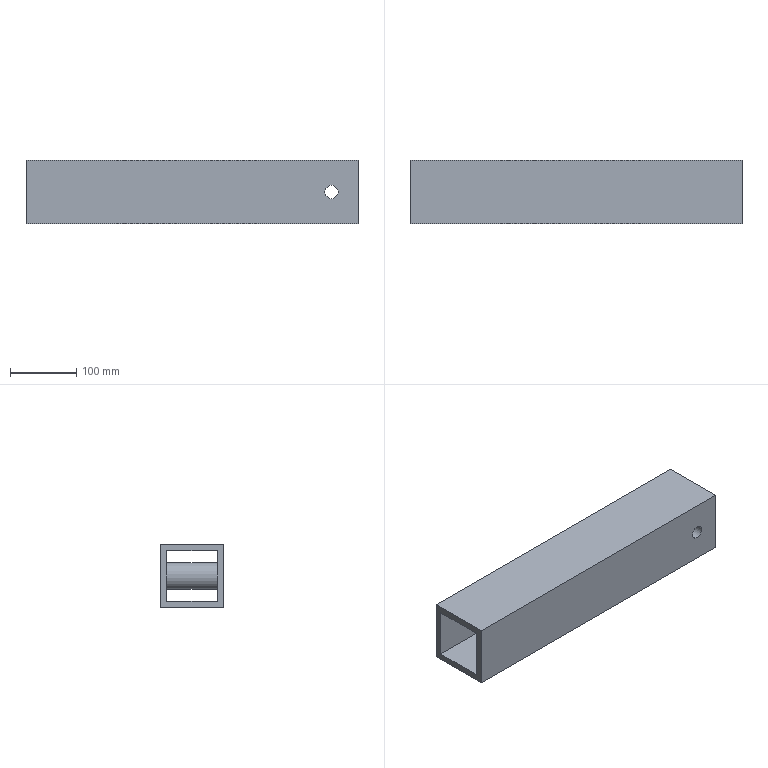Component | NX | TELESCOPIC_ROD | 1 solid | 12 faces | box 500 x 96 x 96 mm | volume 1785345 mm3 | plane 10 | cylinder 2 | commonest cylinder face diameters 20 x1 40 x1
STEP:
#1=CARTESIAN_POINT('',(0.,0.,0.));
#2=DIRECTION('',(0.,0.,1.));
#3=DIRECTION('',(1.,0.,0.));
#4=AXIS2_PLACEMENT_3D('',#1,#2,#3);
#5=CARTESIAN_POINT('',(1094.,88.,-44.));
#6=VERTEX_POINT('',#5);
#7=CARTESIAN_POINT('',(1094.,88.,-120.));
#8=VERTEX_POINT('',#7);
#9=CARTESIAN_POINT('',(1094.,88.,-34.));
#10=DIRECTION('',(0.,-0.,-1.));
#11=VECTOR('',#10,1.);
#12=LINE('',#9,#11);
#13=CARTESIAN_POINT('',(1094.,174.,-34.));
#14=DIRECTION('',(-1.,0.,0.));
#15=DIRECTION('',(0.,-1.,0.));
#16=AXIS2_PLACEMENT_3D('',#13,#14,#15);
#17=PLANE('',#16);
#18=CARTESIAN_POINT('',(86.,0.));
#19=DIRECTION('',(0.,-1.));
#20=VECTOR('',#19,1.);
#21=LINE('',#18,#20);
#22=(GEOMETRIC_REPRESENTATION_CONTEXT(2)PARAMETRIC_REPRESENTATION_CONTEXT()REPRESENTATION_CONTEXT('',''));
#23=DEFINITIONAL_REPRESENTATION('',(#21),#22);
#24=PCURVE('',#17,#23);
#25=CARTESIAN_POINT('',(594.,88.,-34.));
#26=DIRECTION('',(0.,-1.,0.));
#27=DIRECTION('',(0.,-0.,-1.));
#28=AXIS2_PLACEMENT_3D('',#25,#26,#27);
#29=PLANE('',#28);
#30=CARTESIAN_POINT('',(0.,500.));
#31=DIRECTION('',(1.,0.));
#32=VECTOR('',#31,1.);
#33=LINE('',#30,#32);
#34=(GEOMETRIC_REPRESENTATION_CONTEXT(2)PARAMETRIC_REPRESENTATION_CONTEXT()REPRESENTATION_CONTEXT('',''));
#35=DEFINITIONAL_REPRESENTATION('',(#33),#34);
#36=PCURVE('',#29,#35);
#37=SURFACE_CURVE('',#12,(#24,#36),.PCURVE_S1.);
#38=EDGE_CURVE('',#6,#8,#37,.T.);
#39=ORIENTED_EDGE('',*,*,#38,.F.);
#40=CARTESIAN_POINT('',(1094.,164.,-44.));
#41=VERTEX_POINT('',#40);
#42=CARTESIAN_POINT('',(1094.,174.,-44.));
#43=DIRECTION('',(0.,-1.,0.));
#44=VECTOR('',#43,1.);
#45=LINE('',#42,#44);
#46=CARTESIAN_POINT('',(0.,-10.));
#47=DIRECTION('',(1.,0.));
#48=VECTOR('',#47,1.);
#49=LINE('',#46,#48);
#50=(GEOMETRIC_REPRESENTATION_CONTEXT(2)PARAMETRIC_REPRESENTATION_CONTEXT()REPRESENTATION_CONTEXT('',''));
#51=DEFINITIONAL_REPRESENTATION('',(#49),#50);
#52=PCURVE('',#17,#51);
#53=CARTESIAN_POINT('',(594.,174.,-44.));
#54=DIRECTION('',(0.,0.,1.));
#55=DIRECTION('',(1.,0.,0.));
#56=AXIS2_PLACEMENT_3D('',#53,#54,#55);
#57=PLANE('',#56);
#58=CARTESIAN_POINT('',(500.,0.));
#59=DIRECTION('',(0.,-1.));
#60=VECTOR('',#59,1.);
#61=LINE('',#58,#60);
#62=(GEOMETRIC_REPRESENTATION_CONTEXT(2)PARAMETRIC_REPRESENTATION_CONTEXT()REPRESENTATION_CONTEXT('',''));
#63=DEFINITIONAL_REPRESENTATION('',(#61),#62);
#64=PCURVE('',#57,#63);
#65=SURFACE_CURVE('',#45,(#52,#64),.PCURVE_S1.);
#66=EDGE_CURVE('',#41,#6,#65,.T.);
#67=ORIENTED_EDGE('',*,*,#66,.F.);
#68=CARTESIAN_POINT('',(1094.,164.,-120.));
#69=VERTEX_POINT('',#68);
#70=CARTESIAN_POINT('',(1094.,164.,-130.));
#71=DIRECTION('',(0.,-0.,1.));
#72=VECTOR('',#71,1.);
#73=LINE('',#70,#72);
#74=CARTESIAN_POINT('',(10.,-96.));
#75=DIRECTION('',(0.,1.));
#76=VECTOR('',#75,1.);
#77=LINE('',#74,#76);
#78=(GEOMETRIC_REPRESENTATION_CONTEXT(2)PARAMETRIC_REPRESENTATION_CONTEXT()REPRESENTATION_CONTEXT('',''));
#79=DEFINITIONAL_REPRESENTATION('',(#77),#78);
#80=PCURVE('',#17,#79);
#81=CARTESIAN_POINT('',(594.,164.,-130.));
#82=DIRECTION('',(0.,1.,0.));
#83=DIRECTION('',(0.,-0.,1.));
#84=AXIS2_PLACEMENT_3D('',#81,#82,#83);
#85=PLANE('',#84);
#86=CARTESIAN_POINT('',(0.,500.));
#87=DIRECTION('',(1.,0.));
#88=VECTOR('',#87,1.);
#89=LINE('',#86,#88);
#90=(GEOMETRIC_REPRESENTATION_CONTEXT(2)PARAMETRIC_REPRESENTATION_CONTEXT()REPRESENTATION_CONTEXT('',''));
#91=DEFINITIONAL_REPRESENTATION('',(#89),#90);
#92=PCURVE('',#85,#91);
#93=SURFACE_CURVE('',#73,(#80,#92),.PCURVE_S1.);
#94=EDGE_CURVE('',#69,#41,#93,.T.);
#95=ORIENTED_EDGE('',*,*,#94,.F.);
#96=CARTESIAN_POINT('',(1094.,78.,-120.));
#97=DIRECTION('',(0.,1.,0.));
#98=VECTOR('',#97,1.);
#99=LINE('',#96,#98);
#100=CARTESIAN_POINT('',(96.,-86.));
#101=DIRECTION('',(-1.,0.));
#102=VECTOR('',#101,1.);
#103=LINE('',#100,#102);
#104=(GEOMETRIC_REPRESENTATION_CONTEXT(2)PARAMETRIC_REPRESENTATION_CONTEXT()REPRESENTATION_CONTEXT('',''));
#105=DEFINITIONAL_REPRESENTATION('',(#103),#104);
#106=PCURVE('',#17,#105);
#107=CARTESIAN_POINT('',(594.,78.,-120.));
#108=DIRECTION('',(0.,0.,-1.));
#109=DIRECTION('',(-1.,0.,0.));
#110=AXIS2_PLACEMENT_3D('',#107,#108,#109);
#111=PLANE('',#110);
#112=CARTESIAN_POINT('',(-500.,0.));
#113=DIRECTION('',(0.,1.));
#114=VECTOR('',#113,1.);
#115=LINE('',#112,#114);
#116=(GEOMETRIC_REPRESENTATION_CONTEXT(2)PARAMETRIC_REPRESENTATION_CONTEXT()REPRESENTATION_CONTEXT('',''));
#117=DEFINITIONAL_REPRESENTATION('',(#115),#116);
#118=PCURVE('',#111,#117);
#119=SURFACE_CURVE('',#99,(#106,#118),.PCURVE_S1.);
#120=EDGE_CURVE('',#8,#69,#119,.T.);
#121=ORIENTED_EDGE('',*,*,#120,.F.);
#122=EDGE_LOOP('',(#39,#67,#95,#121));
#123=FACE_BOUND('',#122,.T.);
#124=CARTESIAN_POINT('',(1094.,174.,-34.));
#125=VERTEX_POINT('',#124);
#126=CARTESIAN_POINT('',(1094.,78.,-34.));
#127=VERTEX_POINT('',#126);
#128=CARTESIAN_POINT('',(1094.,174.,-34.));
#129=DIRECTION('',(0.,-1.,0.));
#130=VECTOR('',#129,1.);
#131=LINE('',#128,#130);
#132=CARTESIAN_POINT('',(0.,0.));
#133=DIRECTION('',(1.,0.));
#134=VECTOR('',#133,1.);
#135=LINE('',#132,#134);
#136=(GEOMETRIC_REPRESENTATION_CONTEXT(2)PARAMETRIC_REPRESENTATION_CONTEXT()REPRESENTATION_CONTEXT('',''));
#137=DEFINITIONAL_REPRESENTATION('',(#135),#136);
#138=PCURVE('',#17,#137);
#139=CARTESIAN_POINT('',(594.,174.,-34.));
#140=DIRECTION('',(0.,0.,1.));
#141=DIRECTION('',(1.,0.,0.));
#142=AXIS2_PLACEMENT_3D('',#139,#140,#141);
#143=PLANE('',#142);
#144=CARTESIAN_POINT('',(500.,0.));
#145=DIRECTION('',(0.,-1.));
#146=VECTOR('',#145,1.);
#147=LINE('',#144,#146);
#148=(GEOMETRIC_REPRESENTATION_CONTEXT(2)PARAMETRIC_REPRESENTATION_CONTEXT()REPRESENTATION_CONTEXT('',''));
#149=DEFINITIONAL_REPRESENTATION('',(#147),#148);
#150=PCURVE('',#143,#149);
#151=SURFACE_CURVE('',#131,(#138,#150),.PCURVE_S1.);
#152=EDGE_CURVE('',#125,#127,#151,.T.);
#153=ORIENTED_EDGE('',*,*,#152,.T.);
#154=CARTESIAN_POINT('',(1094.,78.,-130.));
#155=VERTEX_POINT('',#154);
#156=CARTESIAN_POINT('',(1094.,78.,-34.));
#157=DIRECTION('',(0.,-0.,-1.));
#158=VECTOR('',#157,1.);
#159=LINE('',#156,#158);
#160=CARTESIAN_POINT('',(96.,0.));
#161=DIRECTION('',(0.,-1.));
#162=VECTOR('',#161,1.);
#163=LINE('',#160,#162);
#164=(GEOMETRIC_REPRESENTATION_CONTEXT(2)PARAMETRIC_REPRESENTATION_CONTEXT()REPRESENTATION_CONTEXT('',''));
#165=DEFINITIONAL_REPRESENTATION('',(#163),#164);
#166=PCURVE('',#17,#165);
#167=CARTESIAN_POINT('',(594.,78.,-34.));
#168=DIRECTION('',(0.,-1.,0.));
#169=DIRECTION('',(0.,-0.,-1.));
#170=AXIS2_PLACEMENT_3D('',#167,#168,#169);
#171=PLANE('',#170);
#172=CARTESIAN_POINT('',(0.,500.));
#173=DIRECTION('',(1.,0.));
#174=VECTOR('',#173,1.);
#175=LINE('',#172,#174);
#176=(GEOMETRIC_REPRESENTATION_CONTEXT(2)PARAMETRIC_REPRESENTATION_CONTEXT()REPRESENTATION_CONTEXT('',''));
#177=DEFINITIONAL_REPRESENTATION('',(#175),#176);
#178=PCURVE('',#171,#177);
#179=SURFACE_CURVE('',#159,(#166,#178),.PCURVE_S1.);
#180=EDGE_CURVE('',#127,#155,#179,.T.);
#181=ORIENTED_EDGE('',*,*,#180,.T.);
#182=CARTESIAN_POINT('',(1094.,174.,-130.));
#183=VERTEX_POINT('',#182);
#184=CARTESIAN_POINT('',(1094.,78.,-130.));
#185=DIRECTION('',(0.,1.,0.));
#186=VECTOR('',#185,1.);
#187=LINE('',#184,#186);
#188=CARTESIAN_POINT('',(96.,-96.));
#189=DIRECTION('',(-1.,0.));
#190=VECTOR('',#189,1.);
#191=LINE('',#188,#190);
#192=(GEOMETRIC_REPRESENTATION_CONTEXT(2)PARAMETRIC_REPRESENTATION_CONTEXT()REPRESENTATION_CONTEXT('',''));
#193=DEFINITIONAL_REPRESENTATION('',(#191),#192);
#194=PCURVE('',#17,#193);
#195=CARTESIAN_POINT('',(594.,78.,-130.));
#196=DIRECTION('',(0.,0.,-1.));
#197=DIRECTION('',(-1.,0.,0.));
#198=AXIS2_PLACEMENT_3D('',#195,#196,#197);
#199=PLANE('',#198);
#200=CARTESIAN_POINT('',(-500.,0.));
#201=DIRECTION('',(0.,1.));
#202=VECTOR('',#201,1.);
#203=LINE('',#200,#202);
#204=(GEOMETRIC_REPRESENTATION_CONTEXT(2)PARAMETRIC_REPRESENTATION_CONTEXT()REPRESENTATION_CONTEXT('',''));
#205=DEFINITIONAL_REPRESENTATION('',(#203),#204);
#206=PCURVE('',#199,#205);
#207=SURFACE_CURVE('',#187,(#194,#206),.PCURVE_S1.);
#208=EDGE_CURVE('',#155,#183,#207,.T.);
#209=ORIENTED_EDGE('',*,*,#208,.T.);
#210=CARTESIAN_POINT('',(1094.,174.,-130.));
#211=DIRECTION('',(0.,-0.,1.));
#212=VECTOR('',#211,1.);
#213=LINE('',#210,#212);
#214=CARTESIAN_POINT('',(0.,-96.));
#215=DIRECTION('',(0.,1.));
#216=VECTOR('',#215,1.);
#217=LINE('',#214,#216);
#218=(GEOMETRIC_REPRESENTATION_CONTEXT(2)PARAMETRIC_REPRESENTATION_CONTEXT()REPRESENTATION_CONTEXT('',''));
#219=DEFINITIONAL_REPRESENTATION('',(#217),#218);
#220=PCURVE('',#17,#219);
#221=CARTESIAN_POINT('',(594.,174.,-130.));
#222=DIRECTION('',(0.,1.,0.));
#223=DIRECTION('',(0.,-0.,1.));
#224=AXIS2_PLACEMENT_3D('',#221,#222,#223);
#225=PLANE('',#224);
#226=CARTESIAN_POINT('',(0.,500.));
#227=DIRECTION('',(1.,0.));
#228=VECTOR('',#227,1.);
#229=LINE('',#226,#228);
#230=(GEOMETRIC_REPRESENTATION_CONTEXT(2)PARAMETRIC_REPRESENTATION_CONTEXT()REPRESENTATION_CONTEXT('',''));
#231=DEFINITIONAL_REPRESENTATION('',(#229),#230);
#232=PCURVE('',#225,#231);
#233=SURFACE_CURVE('',#213,(#220,#232),.PCURVE_S1.);
#234=EDGE_CURVE('',#183,#125,#233,.T.);
#235=ORIENTED_EDGE('',*,*,#234,.T.);
#236=EDGE_LOOP('',(#153,#181,#209,#235));
#237=FACE_BOUND('',#236,.T.);
#238=ADVANCED_FACE('',(#123,#237),#17,.F.);
#239=CARTESIAN_POINT('',(594.,88.,-44.));
#240=VERTEX_POINT('',#239);
#241=CARTESIAN_POINT('',(594.,88.,-120.));
#242=VERTEX_POINT('',#241);
#243=CARTESIAN_POINT('',(594.,88.,-34.));
#244=DIRECTION('',(0.,-0.,-1.));
#245=VECTOR('',#244,1.);
#246=LINE('',#243,#245);
#247=CARTESIAN_POINT('',(594.,78.,-130.));
#248=DIRECTION('',(-1.,0.,0.));
#249=DIRECTION('',(0.,1.,0.));
#250=AXIS2_PLACEMENT_3D('',#247,#248,#249);
#251=PLANE('',#250);
#252=CARTESIAN_POINT('',(10.,-96.));
#253=DIRECTION('',(-0.,1.));
#254=VECTOR('',#253,1.);
#255=LINE('',#252,#254);
#256=(GEOMETRIC_REPRESENTATION_CONTEXT(2)PARAMETRIC_REPRESENTATION_CONTEXT()REPRESENTATION_CONTEXT('',''));
#257=DEFINITIONAL_REPRESENTATION('',(#255),#256);
#258=PCURVE('',#251,#257);
#259=CARTESIAN_POINT('',(0.,0.));
#260=DIRECTION('',(1.,0.));
#261=VECTOR('',#260,1.);
#262=LINE('',#259,#261);
#263=(GEOMETRIC_REPRESENTATION_CONTEXT(2)PARAMETRIC_REPRESENTATION_CONTEXT()REPRESENTATION_CONTEXT('',''));
#264=DEFINITIONAL_REPRESENTATION('',(#262),#263);
#265=PCURVE('',#29,#264);
#266=SURFACE_CURVE('',#246,(#258,#265),.PCURVE_S1.);
#267=EDGE_CURVE('',#240,#242,#266,.T.);
#268=ORIENTED_EDGE('',*,*,#267,.T.);
#269=CARTESIAN_POINT('',(594.,164.,-120.));
#270=VERTEX_POINT('',#269);
#271=CARTESIAN_POINT('',(594.,78.,-120.));
#272=DIRECTION('',(0.,1.,0.));
#273=VECTOR('',#272,1.);
#274=LINE('',#271,#273);
#275=CARTESIAN_POINT('',(0.,-10.));
#276=DIRECTION('',(1.,0.));
#277=VECTOR('',#276,1.);
#278=LINE('',#275,#277);
#279=(GEOMETRIC_REPRESENTATION_CONTEXT(2)PARAMETRIC_REPRESENTATION_CONTEXT()REPRESENTATION_CONTEXT('',''));
#280=DEFINITIONAL_REPRESENTATION('',(#278),#279);
#281=PCURVE('',#251,#280);
#282=CARTESIAN_POINT('',(0.,0.));
#283=DIRECTION('',(0.,1.));
#284=VECTOR('',#283,1.);
#285=LINE('',#282,#284);
#286=(GEOMETRIC_REPRESENTATION_CONTEXT(2)PARAMETRIC_REPRESENTATION_CONTEXT()REPRESENTATION_CONTEXT('',''));
#287=DEFINITIONAL_REPRESENTATION('',(#285),#286);
#288=PCURVE('',#111,#287);
#289=SURFACE_CURVE('',#274,(#281,#288),.PCURVE_S1.);
#290=EDGE_CURVE('',#242,#270,#289,.T.);
#291=ORIENTED_EDGE('',*,*,#290,.T.);
#292=CARTESIAN_POINT('',(594.,164.,-44.));
#293=VERTEX_POINT('',#292);
#294=CARTESIAN_POINT('',(594.,164.,-130.));
#295=DIRECTION('',(0.,-0.,1.));
#296=VECTOR('',#295,1.);
#297=LINE('',#294,#296);
#298=CARTESIAN_POINT('',(86.,0.));
#299=DIRECTION('',(-0.,-1.));
#300=VECTOR('',#299,1.);
#301=LINE('',#298,#300);
#302=(GEOMETRIC_REPRESENTATION_CONTEXT(2)PARAMETRIC_REPRESENTATION_CONTEXT()REPRESENTATION_CONTEXT('',''));
#303=DEFINITIONAL_REPRESENTATION('',(#301),#302);
#304=PCURVE('',#251,#303);
#305=CARTESIAN_POINT('',(0.,0.));
#306=DIRECTION('',(1.,0.));
#307=VECTOR('',#306,1.);
#308=LINE('',#305,#307);
#309=(GEOMETRIC_REPRESENTATION_CONTEXT(2)PARAMETRIC_REPRESENTATION_CONTEXT()REPRESENTATION_CONTEXT('',''));
#310=DEFINITIONAL_REPRESENTATION('',(#308),#309);
#311=PCURVE('',#85,#310);
#312=SURFACE_CURVE('',#297,(#304,#311),.PCURVE_S1.);
#313=EDGE_CURVE('',#270,#293,#312,.T.);
#314=ORIENTED_EDGE('',*,*,#313,.T.);
#315=CARTESIAN_POINT('',(594.,174.,-44.));
#316=DIRECTION('',(0.,-1.,0.));
#317=VECTOR('',#316,1.);
#318=LINE('',#315,#317);
#319=CARTESIAN_POINT('',(96.,-86.));
#320=DIRECTION('',(-1.,0.));
#321=VECTOR('',#320,1.);
#322=LINE('',#319,#321);
#323=(GEOMETRIC_REPRESENTATION_CONTEXT(2)PARAMETRIC_REPRESENTATION_CONTEXT()REPRESENTATION_CONTEXT('',''));
#324=DEFINITIONAL_REPRESENTATION('',(#322),#323);
#325=PCURVE('',#251,#324);
#326=CARTESIAN_POINT('',(0.,0.));
#327=DIRECTION('',(0.,-1.));
#328=VECTOR('',#327,1.);
#329=LINE('',#326,#328);
#330=(GEOMETRIC_REPRESENTATION_CONTEXT(2)PARAMETRIC_REPRESENTATION_CONTEXT()REPRESENTATION_CONTEXT('',''));
#331=DEFINITIONAL_REPRESENTATION('',(#329),#330);
#332=PCURVE('',#57,#331);
#333=SURFACE_CURVE('',#318,(#325,#332),.PCURVE_S1.);
#334=EDGE_CURVE('',#293,#240,#333,.T.);
#335=ORIENTED_EDGE('',*,*,#334,.T.);
#336=EDGE_LOOP('',(#268,#291,#314,#335));
#337=FACE_BOUND('',#336,.T.);
#338=CARTESIAN_POINT('',(594.,78.,-130.));
#339=VERTEX_POINT('',#338);
#340=CARTESIAN_POINT('',(594.,174.,-130.));
#341=VERTEX_POINT('',#340);
#342=CARTESIAN_POINT('',(594.,78.,-130.));
#343=DIRECTION('',(0.,1.,0.));
#344=VECTOR('',#343,1.);
#345=LINE('',#342,#344);
#346=CARTESIAN_POINT('',(0.,0.));
#347=DIRECTION('',(1.,0.));
#348=VECTOR('',#347,1.);
#349=LINE('',#346,#348);
#350=(GEOMETRIC_REPRESENTATION_CONTEXT(2)PARAMETRIC_REPRESENTATION_CONTEXT()REPRESENTATION_CONTEXT('',''));
#351=DEFINITIONAL_REPRESENTATION('',(#349),#350);
#352=PCURVE('',#251,#351);
#353=CARTESIAN_POINT('',(0.,0.));
#354=DIRECTION('',(0.,1.));
#355=VECTOR('',#354,1.);
#356=LINE('',#353,#355);
#357=(GEOMETRIC_REPRESENTATION_CONTEXT(2)PARAMETRIC_REPRESENTATION_CONTEXT()REPRESENTATION_CONTEXT('',''));
#358=DEFINITIONAL_REPRESENTATION('',(#356),#357);
#359=PCURVE('',#199,#358);
#360=SURFACE_CURVE('',#345,(#352,#359),.PCURVE_S1.);
#361=EDGE_CURVE('',#339,#341,#360,.T.);
#362=ORIENTED_EDGE('',*,*,#361,.F.);
#363=CARTESIAN_POINT('',(594.,78.,-34.));
#364=VERTEX_POINT('',#363);
#365=CARTESIAN_POINT('',(594.,78.,-34.));
#366=DIRECTION('',(0.,-0.,-1.));
#367=VECTOR('',#366,1.);
#368=LINE('',#365,#367);
#369=CARTESIAN_POINT('',(0.,-96.));
#370=DIRECTION('',(-0.,1.));
#371=VECTOR('',#370,1.);
#372=LINE('',#369,#371);
#373=(GEOMETRIC_REPRESENTATION_CONTEXT(2)PARAMETRIC_REPRESENTATION_CONTEXT()REPRESENTATION_CONTEXT('',''));
#374=DEFINITIONAL_REPRESENTATION('',(#372),#373);
#375=PCURVE('',#251,#374);
#376=CARTESIAN_POINT('',(0.,0.));
#377=DIRECTION('',(1.,0.));
#378=VECTOR('',#377,1.);
#379=LINE('',#376,#378);
#380=(GEOMETRIC_REPRESENTATION_CONTEXT(2)PARAMETRIC_REPRESENTATION_CONTEXT()REPRESENTATION_CONTEXT('',''));
#381=DEFINITIONAL_REPRESENTATION('',(#379),#380);
#382=PCURVE('',#171,#381);
#383=SURFACE_CURVE('',#368,(#375,#382),.PCURVE_S1.);
#384=EDGE_CURVE('',#364,#339,#383,.T.);
#385=ORIENTED_EDGE('',*,*,#384,.F.);
#386=CARTESIAN_POINT('',(594.,174.,-34.));
#387=VERTEX_POINT('',#386);
#388=CARTESIAN_POINT('',(594.,174.,-34.));
#389=DIRECTION('',(0.,-1.,0.));
#390=VECTOR('',#389,1.);
#391=LINE('',#388,#390);
#392=CARTESIAN_POINT('',(96.,-96.));
#393=DIRECTION('',(-1.,0.));
#394=VECTOR('',#393,1.);
#395=LINE('',#392,#394);
#396=(GEOMETRIC_REPRESENTATION_CONTEXT(2)PARAMETRIC_REPRESENTATION_CONTEXT()REPRESENTATION_CONTEXT('',''));
#397=DEFINITIONAL_REPRESENTATION('',(#395),#396);
#398=PCURVE('',#251,#397);
#399=CARTESIAN_POINT('',(0.,0.));
#400=DIRECTION('',(0.,-1.));
#401=VECTOR('',#400,1.);
#402=LINE('',#399,#401);
#403=(GEOMETRIC_REPRESENTATION_CONTEXT(2)PARAMETRIC_REPRESENTATION_CONTEXT()REPRESENTATION_CONTEXT('',''));
#404=DEFINITIONAL_REPRESENTATION('',(#402),#403);
#405=PCURVE('',#143,#404);
#406=SURFACE_CURVE('',#391,(#398,#405),.PCURVE_S1.);
#407=EDGE_CURVE('',#387,#364,#406,.T.);
#408=ORIENTED_EDGE('',*,*,#407,.F.);
#409=CARTESIAN_POINT('',(594.,174.,-130.));
#410=DIRECTION('',(0.,-0.,1.));
#411=VECTOR('',#410,1.);
#412=LINE('',#409,#411);
#413=CARTESIAN_POINT('',(96.,0.));
#414=DIRECTION('',(-0.,-1.));
#415=VECTOR('',#414,1.);
#416=LINE('',#413,#415);
#417=(GEOMETRIC_REPRESENTATION_CONTEXT(2)PARAMETRIC_REPRESENTATION_CONTEXT()REPRESENTATION_CONTEXT('',''));
#418=DEFINITIONAL_REPRESENTATION('',(#416),#417);
#419=PCURVE('',#251,#418);
#420=CARTESIAN_POINT('',(0.,0.));
#421=DIRECTION('',(1.,0.));
#422=VECTOR('',#421,1.);
#423=LINE('',#420,#422);
#424=(GEOMETRIC_REPRESENTATION_CONTEXT(2)PARAMETRIC_REPRESENTATION_CONTEXT()REPRESENTATION_CONTEXT('',''));
#425=DEFINITIONAL_REPRESENTATION('',(#423),#424);
#426=PCURVE('',#225,#425);
#427=SURFACE_CURVE('',#412,(#419,#426),.PCURVE_S1.);
#428=EDGE_CURVE('',#341,#387,#427,.T.);
#429=ORIENTED_EDGE('',*,*,#428,.F.);
#430=EDGE_LOOP('',(#362,#385,#408,#429));
#431=FACE_BOUND('',#430,.T.);
#432=ADVANCED_FACE('',(#337,#431),#251,.T.);
#433=CARTESIAN_POINT('',(1054.,88.,-62.));
#434=VERTEX_POINT('',#433);
#435=CARTESIAN_POINT('',(1054.,88.,-82.));
#436=DIRECTION('',(0.,-1.,-0.));
#437=DIRECTION('',(0.,-0.,1.));
#438=AXIS2_PLACEMENT_3D('',#435,#436,#437);
#439=CIRCLE('',#438,20.);
#440=CARTESIAN_POINT('',(48.,460.));
#441=DIRECTION('',(-1.,0.));
#442=AXIS2_PLACEMENT_2D('',#440,#441);
#443=CIRCLE('',#442,20.);
#444=(GEOMETRIC_REPRESENTATION_CONTEXT(2)PARAMETRIC_REPRESENTATION_CONTEXT()REPRESENTATION_CONTEXT('',''));
#445=DEFINITIONAL_REPRESENTATION('',(#443),#444);
#446=PCURVE('',#29,#445);
#447=CARTESIAN_POINT('',(1054.,88.,-82.));
#448=DIRECTION('',(0.,1.,0.));
#449=DIRECTION('',(0.,-0.,1.));
#450=AXIS2_PLACEMENT_3D('',#447,#448,#449);
#451=CYLINDRICAL_SURFACE('',#450,20.);
#452=CARTESIAN_POINT('',(6.283,0.));
#453=DIRECTION('',(-1.,0.));
#454=VECTOR('',#453,1.);
#455=LINE('',#452,#454);
#456=(GEOMETRIC_REPRESENTATION_CONTEXT(2)PARAMETRIC_REPRESENTATION_CONTEXT()REPRESENTATION_CONTEXT('',''));
#457=DEFINITIONAL_REPRESENTATION('',(#455),#456);
#458=PCURVE('',#451,#457);
#459=SURFACE_CURVE('',#439,(#446,#458),.PCURVE_S1.);
#460=EDGE_CURVE('',#434,#434,#459,.T.);
#461=ORIENTED_EDGE('',*,*,#460,.T.);
#462=EDGE_LOOP('',(#461));
#463=FACE_BOUND('',#462,.T.);
#464=ORIENTED_EDGE('',*,*,#38,.T.);
#465=CARTESIAN_POINT('',(594.,88.,-120.));
#466=DIRECTION('',(1.,0.,0.));
#467=VECTOR('',#466,1.);
#468=LINE('',#465,#467);
#469=CARTESIAN_POINT('',(86.,0.));
#470=DIRECTION('',(0.,1.));
#471=VECTOR('',#470,1.);
#472=LINE('',#469,#471);
#473=(GEOMETRIC_REPRESENTATION_CONTEXT(2)PARAMETRIC_REPRESENTATION_CONTEXT()REPRESENTATION_CONTEXT('',''));
#474=DEFINITIONAL_REPRESENTATION('',(#472),#473);
#475=PCURVE('',#29,#474);
#476=CARTESIAN_POINT('',(0.,10.));
#477=DIRECTION('',(-1.,0.));
#478=VECTOR('',#477,1.);
#479=LINE('',#476,#478);
#480=(GEOMETRIC_REPRESENTATION_CONTEXT(2)PARAMETRIC_REPRESENTATION_CONTEXT()REPRESENTATION_CONTEXT('',''));
#481=DEFINITIONAL_REPRESENTATION('',(#479),#480);
#482=PCURVE('',#111,#481);
#483=SURFACE_CURVE('',#468,(#475,#482),.PCURVE_S1.);
#484=EDGE_CURVE('',#242,#8,#483,.T.);
#485=ORIENTED_EDGE('',*,*,#484,.F.);
#486=ORIENTED_EDGE('',*,*,#267,.F.);
#487=CARTESIAN_POINT('',(594.,88.,-44.));
#488=DIRECTION('',(1.,0.,0.));
#489=VECTOR('',#488,1.);
#490=LINE('',#487,#489);
#491=CARTESIAN_POINT('',(10.,0.));
#492=DIRECTION('',(0.,1.));
#493=VECTOR('',#492,1.);
#494=LINE('',#491,#493);
#495=(GEOMETRIC_REPRESENTATION_CONTEXT(2)PARAMETRIC_REPRESENTATION_CONTEXT()REPRESENTATION_CONTEXT('',''));
#496=DEFINITIONAL_REPRESENTATION('',(#494),#495);
#497=PCURVE('',#29,#496);
#498=CARTESIAN_POINT('',(0.,-86.));
#499=DIRECTION('',(1.,0.));
#500=VECTOR('',#499,1.);
#501=LINE('',#498,#500);
#502=(GEOMETRIC_REPRESENTATION_CONTEXT(2)PARAMETRIC_REPRESENTATION_CONTEXT()REPRESENTATION_CONTEXT('',''));
#503=DEFINITIONAL_REPRESENTATION('',(#501),#502);
#504=PCURVE('',#57,#503);
#505=SURFACE_CURVE('',#490,(#497,#504),.PCURVE_S1.);
#506=EDGE_CURVE('',#240,#6,#505,.T.);
#507=ORIENTED_EDGE('',*,*,#506,.T.);
#508=EDGE_LOOP('',(#464,#485,#486,#507));
#509=FACE_BOUND('',#508,.T.);
#510=ADVANCED_FACE('',(#463,#509),#29,.F.);
#511=ORIENTED_EDGE('',*,*,#120,.T.);
#512=CARTESIAN_POINT('',(594.,164.,-120.));
#513=DIRECTION('',(1.,0.,0.));
#514=VECTOR('',#513,1.);
#515=LINE('',#512,#514);
#516=CARTESIAN_POINT('',(0.,86.));
#517=DIRECTION('',(-1.,0.));
#518=VECTOR('',#517,1.);
#519=LINE('',#516,#518);
#520=(GEOMETRIC_REPRESENTATION_CONTEXT(2)PARAMETRIC_REPRESENTATION_CONTEXT()REPRESENTATION_CONTEXT('',''));
#521=DEFINITIONAL_REPRESENTATION('',(#519),#520);
#522=PCURVE('',#111,#521);
#523=CARTESIAN_POINT('',(10.,0.));
#524=DIRECTION('',(0.,1.));
#525=VECTOR('',#524,1.);
#526=LINE('',#523,#525);
#527=(GEOMETRIC_REPRESENTATION_CONTEXT(2)PARAMETRIC_REPRESENTATION_CONTEXT()REPRESENTATION_CONTEXT('',''));
#528=DEFINITIONAL_REPRESENTATION('',(#526),#527);
#529=PCURVE('',#85,#528);
#530=SURFACE_CURVE('',#515,(#522,#529),.PCURVE_S1.);
#531=EDGE_CURVE('',#270,#69,#530,.T.);
#532=ORIENTED_EDGE('',*,*,#531,.F.);
#533=ORIENTED_EDGE('',*,*,#290,.F.);
#534=ORIENTED_EDGE('',*,*,#484,.T.);
#535=EDGE_LOOP('',(#511,#532,#533,#534));
#536=FACE_BOUND('',#535,.T.);
#537=ADVANCED_FACE('',(#536),#111,.F.);
#538=CARTESIAN_POINT('',(1054.,164.,-62.));
#539=VERTEX_POINT('',#538);
#540=CARTESIAN_POINT('',(1054.,164.,-82.));
#541=DIRECTION('',(0.,1.,0.));
#542=DIRECTION('',(0.,-0.,1.));
#543=AXIS2_PLACEMENT_3D('',#540,#541,#542);
#544=CIRCLE('',#543,20.);
#545=CARTESIAN_POINT('',(48.,460.));
#546=DIRECTION('',(1.,0.));
#547=AXIS2_PLACEMENT_2D('',#545,#546);
#548=CIRCLE('',#547,20.);
#549=(GEOMETRIC_REPRESENTATION_CONTEXT(2)PARAMETRIC_REPRESENTATION_CONTEXT()REPRESENTATION_CONTEXT('',''));
#550=DEFINITIONAL_REPRESENTATION('',(#548),#549);
#551=PCURVE('',#85,#550);
#552=CARTESIAN_POINT('',(0.,76.));
#553=DIRECTION('',(1.,0.));
#554=VECTOR('',#553,1.);
#555=LINE('',#552,#554);
#556=(GEOMETRIC_REPRESENTATION_CONTEXT(2)PARAMETRIC_REPRESENTATION_CONTEXT()REPRESENTATION_CONTEXT('',''));
#557=DEFINITIONAL_REPRESENTATION('',(#555),#556);
#558=PCURVE('',#451,#557);
#559=SURFACE_CURVE('',#544,(#551,#558),.PCURVE_S1.);
#560=EDGE_CURVE('',#539,#539,#559,.T.);
#561=ORIENTED_EDGE('',*,*,#560,.T.);
#562=EDGE_LOOP('',(#561));
#563=FACE_BOUND('',#562,.T.);
#564=ORIENTED_EDGE('',*,*,#94,.T.);
#565=CARTESIAN_POINT('',(594.,164.,-44.));
#566=DIRECTION('',(1.,0.,0.));
#567=VECTOR('',#566,1.);
#568=LINE('',#565,#567);
#569=CARTESIAN_POINT('',(86.,0.));
#570=DIRECTION('',(0.,1.));
#571=VECTOR('',#570,1.);
#572=LINE('',#569,#571);
#573=(GEOMETRIC_REPRESENTATION_CONTEXT(2)PARAMETRIC_REPRESENTATION_CONTEXT()REPRESENTATION_CONTEXT('',''));
#574=DEFINITIONAL_REPRESENTATION('',(#572),#573);
#575=PCURVE('',#85,#574);
#576=CARTESIAN_POINT('',(0.,-10.));
#577=DIRECTION('',(1.,0.));
#578=VECTOR('',#577,1.);
#579=LINE('',#576,#578);
#580=(GEOMETRIC_REPRESENTATION_CONTEXT(2)PARAMETRIC_REPRESENTATION_CONTEXT()REPRESENTATION_CONTEXT('',''));
#581=DEFINITIONAL_REPRESENTATION('',(#579),#580);
#582=PCURVE('',#57,#581);
#583=SURFACE_CURVE('',#568,(#575,#582),.PCURVE_S1.);
#584=EDGE_CURVE('',#293,#41,#583,.T.);
#585=ORIENTED_EDGE('',*,*,#584,.F.);
#586=ORIENTED_EDGE('',*,*,#313,.F.);
#587=ORIENTED_EDGE('',*,*,#531,.T.);
#588=EDGE_LOOP('',(#564,#585,#586,#587));
#589=FACE_BOUND('',#588,.T.);
#590=ADVANCED_FACE('',(#563,#589),#85,.F.);
#591=ORIENTED_EDGE('',*,*,#66,.T.);
#592=ORIENTED_EDGE('',*,*,#506,.F.);
#593=ORIENTED_EDGE('',*,*,#334,.F.);
#594=ORIENTED_EDGE('',*,*,#584,.T.);
#595=EDGE_LOOP('',(#591,#592,#593,#594));
#596=FACE_BOUND('',#595,.T.);
#597=ADVANCED_FACE('',(#596),#57,.F.);
#598=CARTESIAN_POINT('',(1054.,78.,-72.));
#599=VERTEX_POINT('',#598);
#600=CARTESIAN_POINT('',(1054.,78.,-82.));
#601=DIRECTION('',(0.,1.,-0.));
#602=DIRECTION('',(0.,0.,1.));
#603=AXIS2_PLACEMENT_3D('',#600,#601,#602);
#604=CIRCLE('',#603,10.);
#605=CARTESIAN_POINT('',(38.,460.));
#606=CARTESIAN_POINT('',(38.,477.321));
#607=CARTESIAN_POINT('',(53.,468.66));
#608=CARTESIAN_POINT('',(68.,460.));
#609=CARTESIAN_POINT('',(53.,451.34));
#610=CARTESIAN_POINT('',(38.,442.679));
#611=CARTESIAN_POINT('',(38.,460.));
#612=(BOUNDED_CURVE()B_SPLINE_CURVE(2,(#605,#606,#607,#608,#609,#610,#611),.UNSPECIFIED.,.T.,.F.)B_SPLINE_CURVE_WITH_KNOTS((1,2,2,2,2,1),(-2.094,0.,2.094,4.189,6.283,8.378),.UNSPECIFIED.)CURVE()GEOMETRIC_REPRESENTATION_ITEM()RATIONAL_B_SPLINE_CURVE((1.,0.5,1.,0.5,1.,0.5,1.))REPRESENTATION_ITEM(''));
#613=(GEOMETRIC_REPRESENTATION_CONTEXT(2)PARAMETRIC_REPRESENTATION_CONTEXT()REPRESENTATION_CONTEXT('',''));
#614=DEFINITIONAL_REPRESENTATION('',(#612),#613);
#615=PCURVE('',#171,#614);
#616=CARTESIAN_POINT('',(1054.,78.,-82.));
#617=DIRECTION('',(0.,1.,-0.));
#618=DIRECTION('',(0.,0.,1.));
#619=AXIS2_PLACEMENT_3D('',#616,#617,#618);
#620=CYLINDRICAL_SURFACE('',#619,10.);
#621=CARTESIAN_POINT('',(0.,0.));
#622=DIRECTION('',(1.,0.));
#623=VECTOR('',#622,1.);
#624=LINE('',#621,#623);
#625=(GEOMETRIC_REPRESENTATION_CONTEXT(2)PARAMETRIC_REPRESENTATION_CONTEXT()REPRESENTATION_CONTEXT('',''));
#626=DEFINITIONAL_REPRESENTATION('',(#624),#625);
#627=PCURVE('',#620,#626);
#628=SURFACE_CURVE('',#604,(#615,#627),.PCURVE_S1.);
#629=EDGE_CURVE('',#599,#599,#628,.T.);
#630=ORIENTED_EDGE('',*,*,#629,.T.);
#631=EDGE_LOOP('',(#630));
#632=FACE_BOUND('',#631,.T.);
#633=ORIENTED_EDGE('',*,*,#180,.F.);
#634=CARTESIAN_POINT('',(594.,78.,-34.));
#635=DIRECTION('',(1.,0.,0.));
#636=VECTOR('',#635,1.);
#637=LINE('',#634,#636);
#638=CARTESIAN_POINT('',(0.,0.));
#639=DIRECTION('',(0.,1.));
#640=VECTOR('',#639,1.);
#641=LINE('',#638,#640);
#642=(GEOMETRIC_REPRESENTATION_CONTEXT(2)PARAMETRIC_REPRESENTATION_CONTEXT()REPRESENTATION_CONTEXT('',''));
#643=DEFINITIONAL_REPRESENTATION('',(#641),#642);
#644=PCURVE('',#171,#643);
#645=CARTESIAN_POINT('',(0.,-96.));
#646=DIRECTION('',(1.,0.));
#647=VECTOR('',#646,1.);
#648=LINE('',#645,#647);
#649=(GEOMETRIC_REPRESENTATION_CONTEXT(2)PARAMETRIC_REPRESENTATION_CONTEXT()REPRESENTATION_CONTEXT('',''));
#650=DEFINITIONAL_REPRESENTATION('',(#648),#649);
#651=PCURVE('',#143,#650);
#652=SURFACE_CURVE('',#637,(#644,#651),.PCURVE_S1.);
#653=EDGE_CURVE('',#364,#127,#652,.T.);
#654=ORIENTED_EDGE('',*,*,#653,.F.);
#655=ORIENTED_EDGE('',*,*,#384,.T.);
#656=CARTESIAN_POINT('',(594.,78.,-130.));
#657=DIRECTION('',(1.,0.,0.));
#658=VECTOR('',#657,1.);
#659=LINE('',#656,#658);
#660=CARTESIAN_POINT('',(96.,0.));
#661=DIRECTION('',(0.,1.));
#662=VECTOR('',#661,1.);
#663=LINE('',#660,#662);
#664=(GEOMETRIC_REPRESENTATION_CONTEXT(2)PARAMETRIC_REPRESENTATION_CONTEXT()REPRESENTATION_CONTEXT('',''));
#665=DEFINITIONAL_REPRESENTATION('',(#663),#664);
#666=PCURVE('',#171,#665);
#667=CARTESIAN_POINT('',(0.,0.));
#668=DIRECTION('',(-1.,0.));
#669=VECTOR('',#668,1.);
#670=LINE('',#667,#669);
#671=(GEOMETRIC_REPRESENTATION_CONTEXT(2)PARAMETRIC_REPRESENTATION_CONTEXT()REPRESENTATION_CONTEXT('',''));
#672=DEFINITIONAL_REPRESENTATION('',(#670),#671);
#673=PCURVE('',#199,#672);
#674=SURFACE_CURVE('',#659,(#666,#673),.PCURVE_S1.);
#675=EDGE_CURVE('',#339,#155,#674,.T.);
#676=ORIENTED_EDGE('',*,*,#675,.T.);
#677=EDGE_LOOP('',(#633,#654,#655,#676));
#678=FACE_BOUND('',#677,.T.);
#679=ADVANCED_FACE('',(#632,#678),#171,.T.);
#680=ORIENTED_EDGE('',*,*,#208,.F.);
#681=ORIENTED_EDGE('',*,*,#675,.F.);
#682=ORIENTED_EDGE('',*,*,#361,.T.);
#683=CARTESIAN_POINT('',(594.,174.,-130.));
#684=DIRECTION('',(1.,0.,0.));
#685=VECTOR('',#684,1.);
#686=LINE('',#683,#685);
#687=CARTESIAN_POINT('',(0.,96.));
#688=DIRECTION('',(-1.,0.));
#689=VECTOR('',#688,1.);
#690=LINE('',#687,#689);
#691=(GEOMETRIC_REPRESENTATION_CONTEXT(2)PARAMETRIC_REPRESENTATION_CONTEXT()REPRESENTATION_CONTEXT('',''));
#692=DEFINITIONAL_REPRESENTATION('',(#690),#691);
#693=PCURVE('',#199,#692);
#694=CARTESIAN_POINT('',(0.,0.));
#695=DIRECTION('',(0.,1.));
#696=VECTOR('',#695,1.);
#697=LINE('',#694,#696);
#698=(GEOMETRIC_REPRESENTATION_CONTEXT(2)PARAMETRIC_REPRESENTATION_CONTEXT()REPRESENTATION_CONTEXT('',''));
#699=DEFINITIONAL_REPRESENTATION('',(#697),#698);
#700=PCURVE('',#225,#699);
#701=SURFACE_CURVE('',#686,(#693,#700),.PCURVE_S1.);
#702=EDGE_CURVE('',#341,#183,#701,.T.);
#703=ORIENTED_EDGE('',*,*,#702,.T.);
#704=EDGE_LOOP('',(#680,#681,#682,#703));
#705=FACE_BOUND('',#704,.T.);
#706=ADVANCED_FACE('',(#705),#199,.T.);
#707=CARTESIAN_POINT('',(1054.,174.,-72.));
#708=VERTEX_POINT('',#707);
#709=CARTESIAN_POINT('',(1054.,174.,-82.));
#710=DIRECTION('',(0.,1.,0.));
#711=DIRECTION('',(0.,-0.,1.));
#712=AXIS2_PLACEMENT_3D('',#709,#710,#711);
#713=CIRCLE('',#712,10.);
#714=CARTESIAN_POINT('',(48.,460.));
#715=DIRECTION('',(1.,0.));
#716=AXIS2_PLACEMENT_2D('',#714,#715);
#717=CIRCLE('',#716,10.);
#718=(GEOMETRIC_REPRESENTATION_CONTEXT(2)PARAMETRIC_REPRESENTATION_CONTEXT()REPRESENTATION_CONTEXT('',''));
#719=DEFINITIONAL_REPRESENTATION('',(#717),#718);
#720=PCURVE('',#225,#719);
#721=CARTESIAN_POINT('',(0.,96.));
#722=DIRECTION('',(1.,0.));
#723=VECTOR('',#722,1.);
#724=LINE('',#721,#723);
#725=(GEOMETRIC_REPRESENTATION_CONTEXT(2)PARAMETRIC_REPRESENTATION_CONTEXT()REPRESENTATION_CONTEXT('',''));
#726=DEFINITIONAL_REPRESENTATION('',(#724),#725);
#727=PCURVE('',#620,#726);
#728=SURFACE_CURVE('',#713,(#720,#727),.PCURVE_S1.);
#729=EDGE_CURVE('',#708,#708,#728,.T.);
#730=ORIENTED_EDGE('',*,*,#729,.F.);
#731=EDGE_LOOP('',(#730));
#732=FACE_BOUND('',#731,.T.);
#733=ORIENTED_EDGE('',*,*,#234,.F.);
#734=ORIENTED_EDGE('',*,*,#702,.F.);
#735=ORIENTED_EDGE('',*,*,#428,.T.);
#736=CARTESIAN_POINT('',(594.,174.,-34.));
#737=DIRECTION('',(1.,0.,0.));
#738=VECTOR('',#737,1.);
#739=LINE('',#736,#738);
#740=CARTESIAN_POINT('',(96.,0.));
#741=DIRECTION('',(0.,1.));
#742=VECTOR('',#741,1.);
#743=LINE('',#740,#742);
#744=(GEOMETRIC_REPRESENTATION_CONTEXT(2)PARAMETRIC_REPRESENTATION_CONTEXT()REPRESENTATION_CONTEXT('',''));
#745=DEFINITIONAL_REPRESENTATION('',(#743),#744);
#746=PCURVE('',#225,#745);
#747=CARTESIAN_POINT('',(0.,0.));
#748=DIRECTION('',(1.,0.));
#749=VECTOR('',#748,1.);
#750=LINE('',#747,#749);
#751=(GEOMETRIC_REPRESENTATION_CONTEXT(2)PARAMETRIC_REPRESENTATION_CONTEXT()REPRESENTATION_CONTEXT('',''));
#752=DEFINITIONAL_REPRESENTATION('',(#750),#751);
#753=PCURVE('',#143,#752);
#754=SURFACE_CURVE('',#739,(#746,#753),.PCURVE_S1.);
#755=EDGE_CURVE('',#387,#125,#754,.T.);
#756=ORIENTED_EDGE('',*,*,#755,.T.);
#757=EDGE_LOOP('',(#733,#734,#735,#756));
#758=FACE_BOUND('',#757,.T.);
#759=ADVANCED_FACE('',(#732,#758),#225,.T.);
#760=ORIENTED_EDGE('',*,*,#152,.F.);
#761=ORIENTED_EDGE('',*,*,#755,.F.);
#762=ORIENTED_EDGE('',*,*,#407,.T.);
#763=ORIENTED_EDGE('',*,*,#653,.T.);
#764=EDGE_LOOP('',(#760,#761,#762,#763));
#765=FACE_BOUND('',#764,.T.);
#766=ADVANCED_FACE('',(#765),#143,.T.);
#767=ORIENTED_EDGE('',*,*,#629,.T.);
#768=CARTESIAN_POINT('',(1054.,78.,-72.));
#769=CARTESIAN_POINT('',(1054.,174.,-72.));
#770=B_SPLINE_CURVE_WITH_KNOTS('',1,(#768,#769),.UNSPECIFIED.,.F.,.F.,(2,2),(0.,96.),.PIECEWISE_BEZIER_KNOTS.);
#771=CARTESIAN_POINT('',(6.283,0.));
#772=DIRECTION('',(0.,1.));
#773=VECTOR('',#772,1.);
#774=LINE('',#771,#773);
#775=(GEOMETRIC_REPRESENTATION_CONTEXT(2)PARAMETRIC_REPRESENTATION_CONTEXT()REPRESENTATION_CONTEXT('',''));
#776=DEFINITIONAL_REPRESENTATION('',(#774),#775);
#777=PCURVE('',#620,#776);
#778=CARTESIAN_POINT('',(0.,0.));
#779=DIRECTION('',(0.,1.));
#780=VECTOR('',#779,1.);
#781=LINE('',#778,#780);
#782=(GEOMETRIC_REPRESENTATION_CONTEXT(2)PARAMETRIC_REPRESENTATION_CONTEXT()REPRESENTATION_CONTEXT('',''));
#783=DEFINITIONAL_REPRESENTATION('',(#781),#782);
#784=PCURVE('',#620,#783);
#785=SEAM_CURVE('',#770,(#777,#784),.PCURVE_S1.);
#786=EDGE_CURVE('',#599,#708,#785,.T.);
#787=ORIENTED_EDGE('',*,*,#786,.T.);
#788=ORIENTED_EDGE('',*,*,#729,.F.);
#789=ORIENTED_EDGE('',*,*,#786,.F.);
#790=EDGE_LOOP('',(#767,#787,#788,#789));
#791=FACE_BOUND('',#790,.F.);
#792=ADVANCED_FACE('',(#791),#620,.F.);
#793=ORIENTED_EDGE('',*,*,#460,.F.);
#794=CARTESIAN_POINT('',(1054.,88.,-62.));
#795=CARTESIAN_POINT('',(1054.,164.,-62.));
#796=B_SPLINE_CURVE_WITH_KNOTS('',1,(#794,#795),.UNSPECIFIED.,.F.,.F.,(2,2),(0.,76.),.PIECEWISE_BEZIER_KNOTS.);
#797=CARTESIAN_POINT('',(6.283,0.));
#798=DIRECTION('',(0.,1.));
#799=VECTOR('',#798,1.);
#800=LINE('',#797,#799);
#801=(GEOMETRIC_REPRESENTATION_CONTEXT(2)PARAMETRIC_REPRESENTATION_CONTEXT()REPRESENTATION_CONTEXT('',''));
#802=DEFINITIONAL_REPRESENTATION('',(#800),#801);
#803=PCURVE('',#451,#802);
#804=CARTESIAN_POINT('',(0.,0.));
#805=DIRECTION('',(0.,1.));
#806=VECTOR('',#805,1.);
#807=LINE('',#804,#806);
#808=(GEOMETRIC_REPRESENTATION_CONTEXT(2)PARAMETRIC_REPRESENTATION_CONTEXT()REPRESENTATION_CONTEXT('',''));
#809=DEFINITIONAL_REPRESENTATION('',(#807),#808);
#810=PCURVE('',#451,#809);
#811=SEAM_CURVE('',#796,(#803,#810),.PCURVE_S1.);
#812=EDGE_CURVE('',#434,#539,#811,.T.);
#813=ORIENTED_EDGE('',*,*,#812,.T.);
#814=ORIENTED_EDGE('',*,*,#560,.F.);
#815=ORIENTED_EDGE('',*,*,#812,.F.);
#816=EDGE_LOOP('',(#793,#813,#814,#815));
#817=FACE_BOUND('',#816,.T.);
#818=ADVANCED_FACE('',(#817),#451,.T.);
#819=CLOSED_SHELL('',(#238,#432,#510,#537,#590,#597,#679,#706,#759,#766,#792,#818));
#820=MANIFOLD_SOLID_BREP('',#819);
#821=(LENGTH_UNIT()NAMED_UNIT(*)SI_UNIT(.MILLI.,.METRE.));
#822=UNCERTAINTY_MEASURE_WITH_UNIT(LENGTH_MEASURE(0.000002),#821,'','');
#823=(NAMED_UNIT(*)PLANE_ANGLE_UNIT()SI_UNIT($,.RADIAN.));
#824=(NAMED_UNIT(*)SI_UNIT($,.STERADIAN.)SOLID_ANGLE_UNIT());
#825=(GEOMETRIC_REPRESENTATION_CONTEXT(3)GLOBAL_UNCERTAINTY_ASSIGNED_CONTEXT((#822))GLOBAL_UNIT_ASSIGNED_CONTEXT((#821,#823,#824))REPRESENTATION_CONTEXT('',''));
#826=ADVANCED_BREP_SHAPE_REPRESENTATION('',(#4,#820),#825);